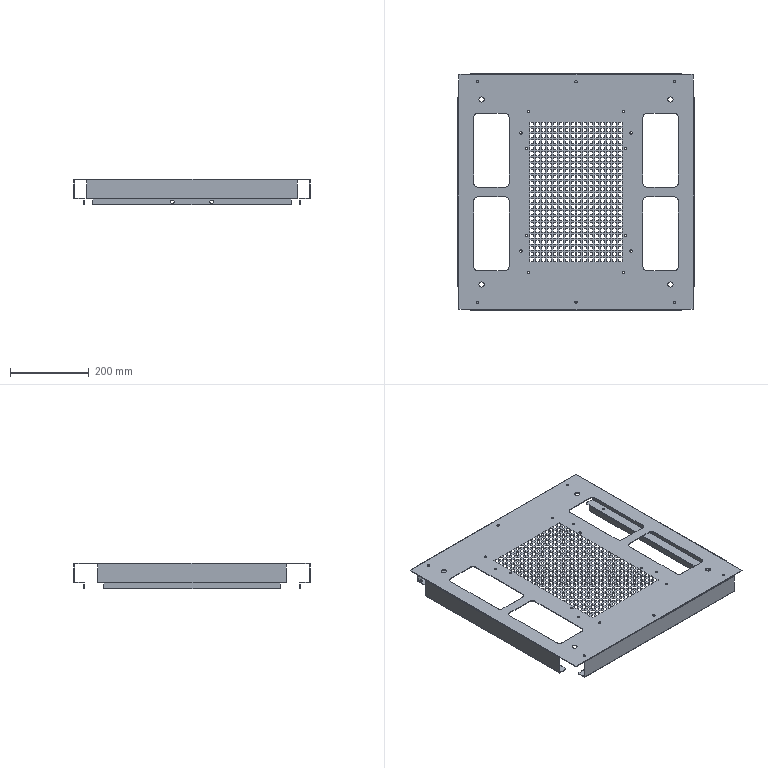Component | SolidWorks | TopBase-1 | 1 solid | 1754 faces | volume 639253 mm3 | plane 1654 | cylinder 100 | commonest cylinder face diameters 6.1 x36 6.5 x16 20 x16 3 x12 9.2 x8 13 x8 2 x4